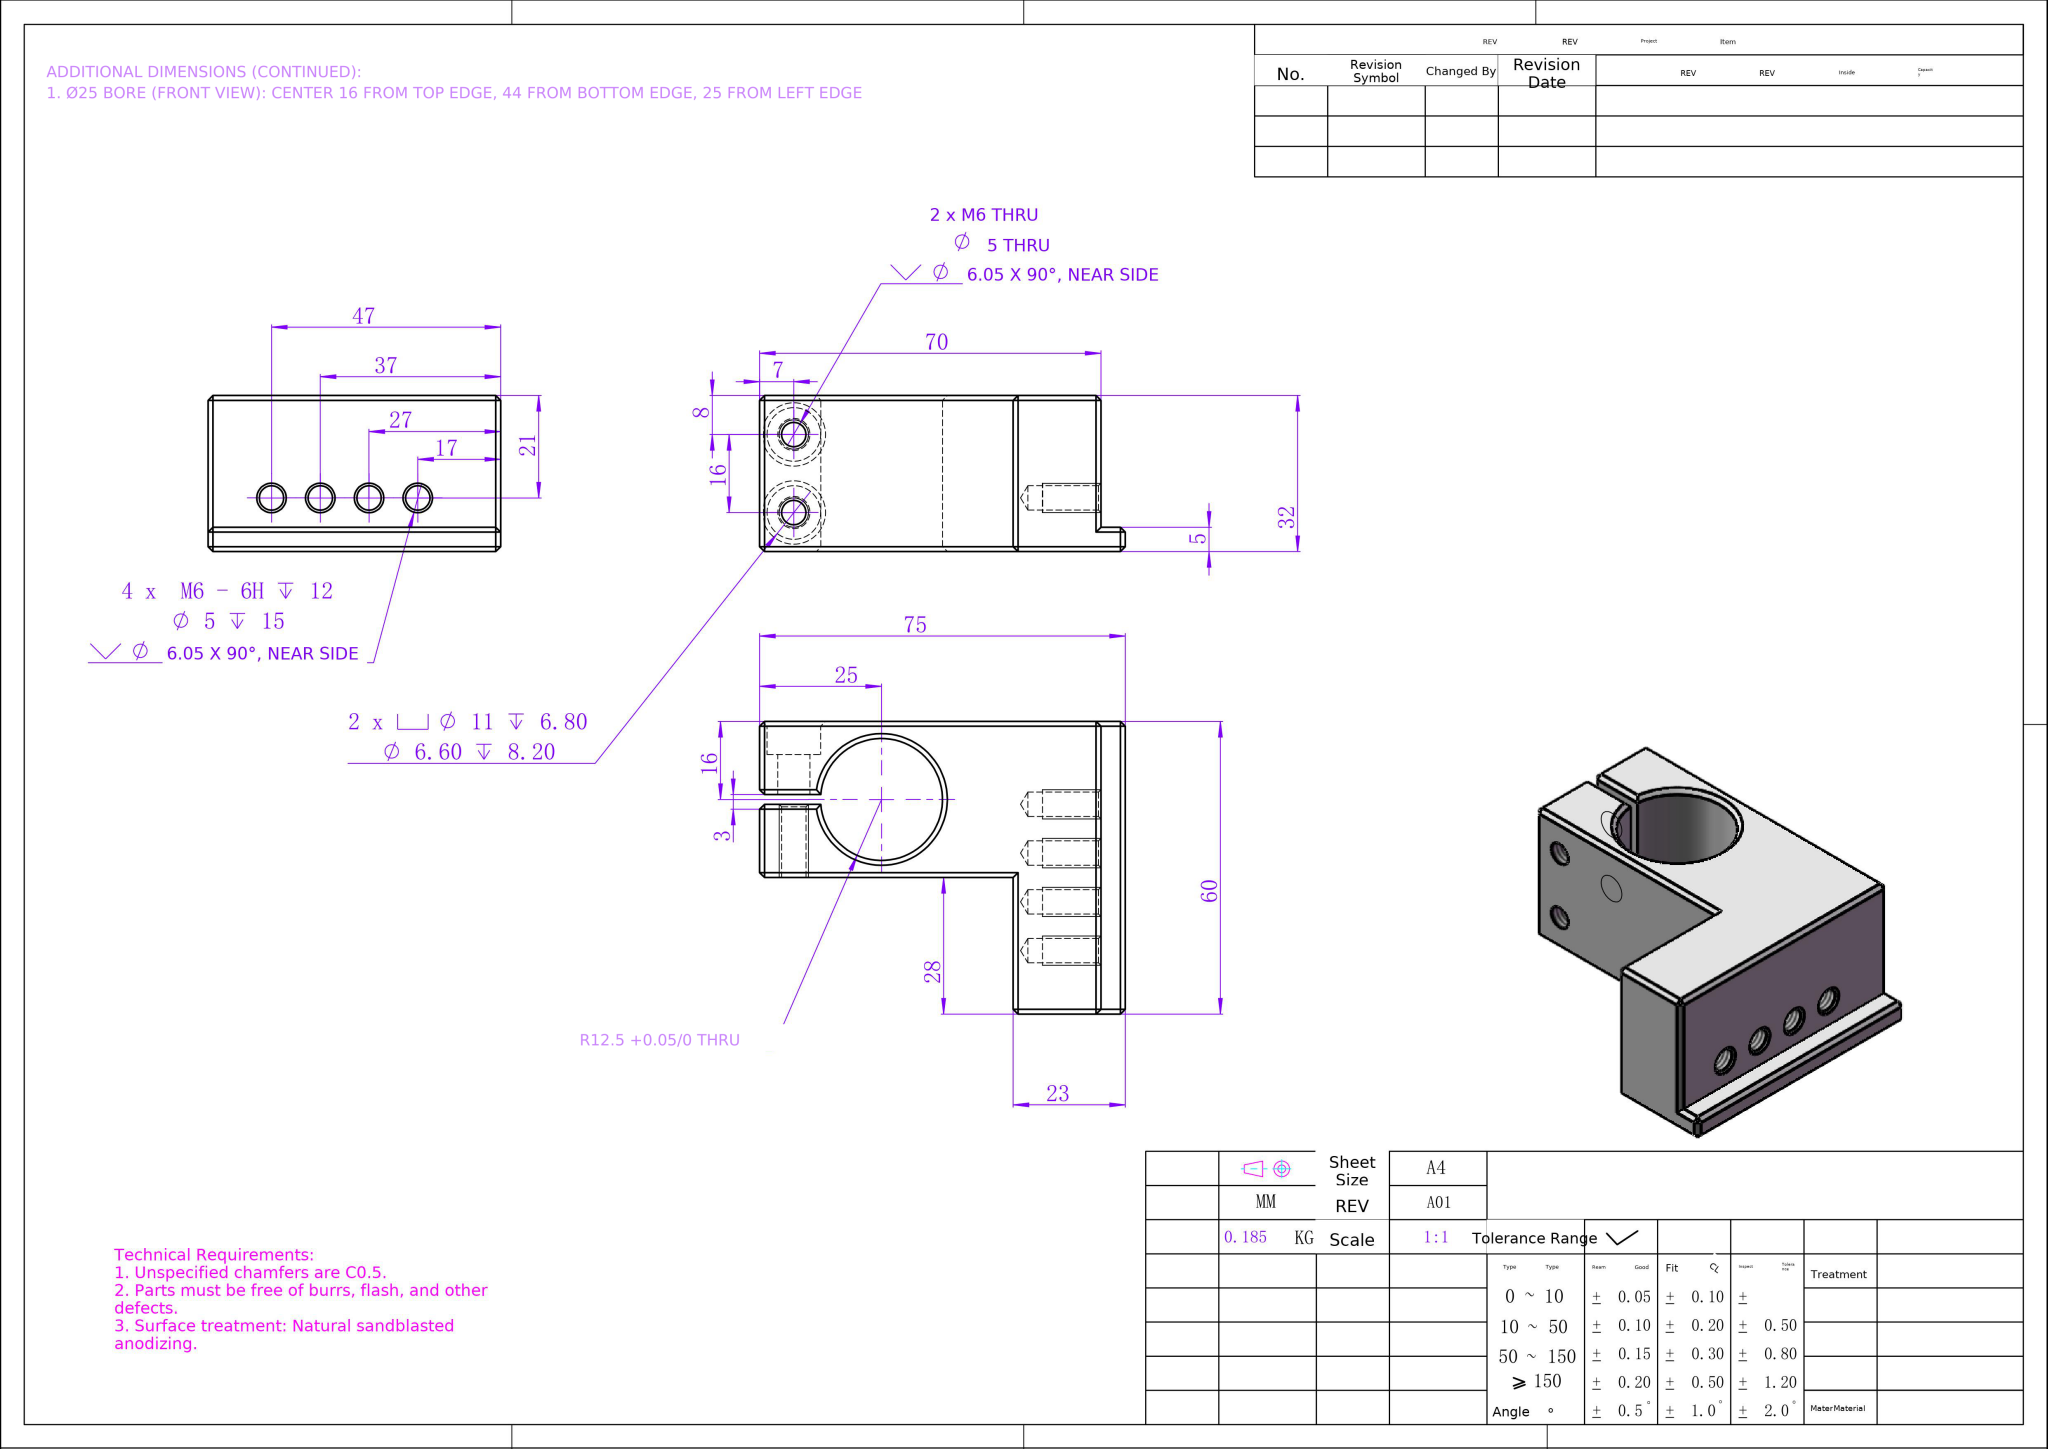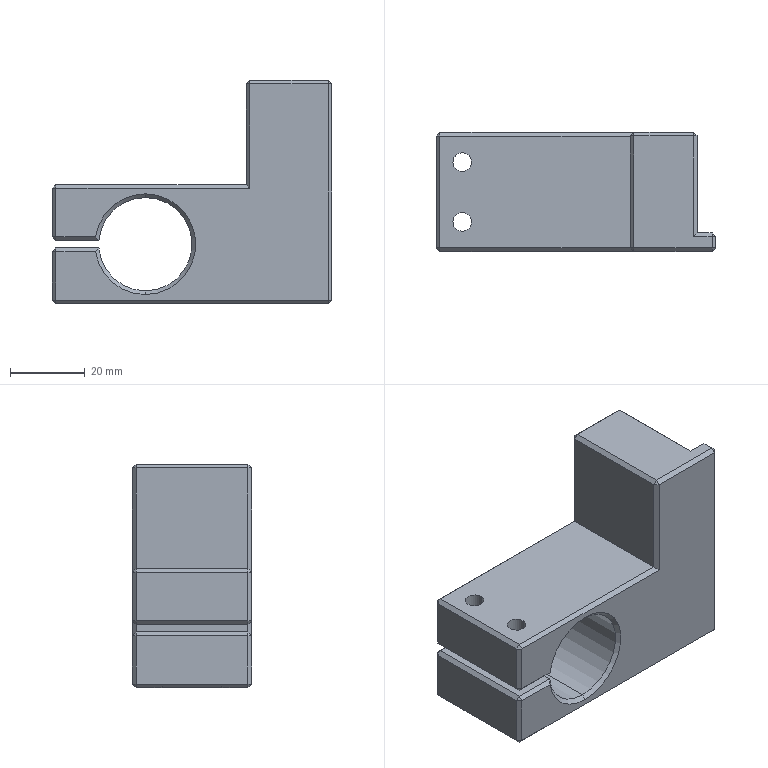Part | NX | mm | 1 solid | 114 faces | box 75 x 32 x 60 mm | volume 68586 mm3 | plane 61 | cone 30 | cylinder 23 | commonest cylinder face diameters 5 x12 6.6 x4 11 x4 25 x3